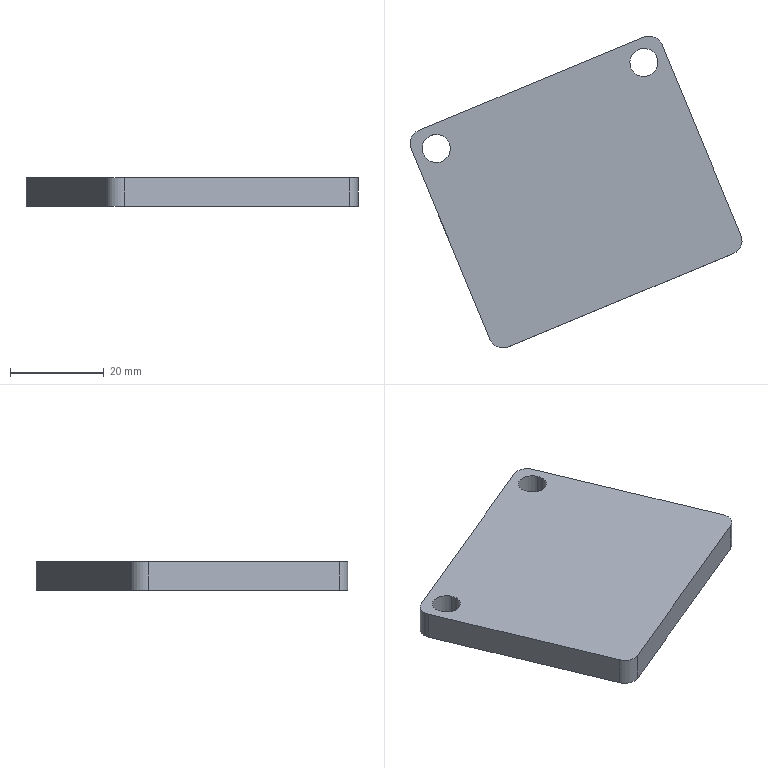Component | SolidWorks | ControlBoard-1 | 1 solid | 14 faces | box 70.89 x 66.56 x 6 mm | volume 17014 mm3 | cylinder 8 | plane 6 | commonest cylinder face diameters 6 x8
build123d program:
from build123d import *

# Parameters (mm, degrees)
SKETCH1_R           = 3
BOSS_EXTRUDE1_DEPTH = 6


with BuildPart() as part:
    # Sketch1 → Boss-Extrude1 (new body)
    with BuildSketch(Plane.XY):
        with BuildLine():
            Line((-18.936, 29.837), (33.064, 29.837))
            ThreePointArc((33.064, 29.837), (35.185, 28.958), (36.064, 26.837))
            Line((36.064, 26.837), (36.064, -17.163))
            ThreePointArc((36.064, -17.163), (35.185, -19.285), (33.064, -20.163))
            Line((33.064, -20.163), (-18.936, -20.163))
            ThreePointArc((-18.936, -20.163), (-21.057, -19.285), (-21.936, -17.163))
            Line((-21.936, -17.163), (-21.936, 26.837))
            ThreePointArc((-21.936, 26.837), (-21.057, 28.958), (-18.936, 29.837))
        make_face()
        with Locations((-16.936, 24.837)):
            Circle(SKETCH1_R, mode=Mode.SUBTRACT)
        with Locations(Location((31.064, 24.837, 0), (0, 0, 180))):
            Circle(SKETCH1_R, mode=Mode.SUBTRACT)
    extrude(amount=BOSS_EXTRUDE1_DEPTH)


solid = part.part

# Placed as in the assembly
solid = solid.moved(Location((28.885, -6.579, 352.846), (0, 0, 22.523)))
STEP:
#1=CARTESIAN_POINT('',(1.783,1.067,14.128));
#2=VERTEX_POINT('',#1);
#3=CARTESIAN_POINT('',(2.001,1.158,14.128));
#4=VERTEX_POINT('',#3);
#5=CARTESIAN_POINT('',(1.892,1.113,14.128));
#6=DIRECTION('',(-0.,0.,1.));
#7=DIRECTION('',(-0.9237,-0.383,0.));
#8=AXIS2_PLACEMENT_3D('',#5,#6,#7);
#9=CIRCLE('',#8,0.1181);
#10=EDGE_CURVE('',#2,#4,#9,.T.);
#11=ORIENTED_EDGE('',*,*,#10,.T.);
#12=CARTESIAN_POINT('',(2.001,1.158,13.892));
#13=VERTEX_POINT('',#12);
#14=CARTESIAN_POINT('',(2.001,1.158,14.128));
#15=DIRECTION('',(0.,-0.,-1.));
#16=VECTOR('',#15,39.37);
#17=LINE('',#14,#16);
#18=EDGE_CURVE('',#4,#13,#17,.T.);
#19=ORIENTED_EDGE('',*,*,#18,.T.);
#20=CARTESIAN_POINT('',(1.783,1.067,13.892));
#21=VERTEX_POINT('',#20);
#22=CARTESIAN_POINT('',(1.892,1.113,13.892));
#23=DIRECTION('',(-0.,0.,1.));
#24=DIRECTION('',(-0.9237,-0.383,0.));
#25=AXIS2_PLACEMENT_3D('',#22,#23,#24);
#26=CIRCLE('',#25,0.1181);
#27=EDGE_CURVE('',#21,#13,#26,.T.);
#28=ORIENTED_EDGE('',*,*,#27,.F.);
#29=CARTESIAN_POINT('',(1.783,1.067,14.128));
#30=DIRECTION('',(0.,-0.,-1.));
#31=VECTOR('',#30,39.37);
#32=LINE('',#29,#31);
#33=EDGE_CURVE('',#2,#21,#32,.T.);
#34=ORIENTED_EDGE('',*,*,#33,.F.);
#35=EDGE_LOOP('',(#11,#19,#28,#34));
#36=FACE_OUTER_BOUND('',#35,.T.);
#37=CARTESIAN_POINT('',(1.892,1.113,14.128));
#38=DIRECTION('',(0.,-0.,-1.));
#39=DIRECTION('',(-0.9237,-0.383,0.));
#40=AXIS2_PLACEMENT_3D('',#37,#38,#39);
#41=CYLINDRICAL_SURFACE('',#40,0.1181);
#42=ADVANCED_FACE('',(#36),#41,.F.);
#43=CARTESIAN_POINT('',(0.03764,0.3436,14.128));
#44=VERTEX_POINT('',#43);
#45=CARTESIAN_POINT('',(0.2558,0.4341,14.128));
#46=VERTEX_POINT('',#45);
#47=CARTESIAN_POINT('',(0.1467,0.3888,14.128));
#48=DIRECTION('',(-0.,0.,1.));
#49=DIRECTION('',(0.9237,0.383,0.));
#50=AXIS2_PLACEMENT_3D('',#47,#48,#49);
#51=CIRCLE('',#50,0.1181);
#52=EDGE_CURVE('',#44,#46,#51,.T.);
#53=ORIENTED_EDGE('',*,*,#52,.T.);
#54=CARTESIAN_POINT('',(0.2558,0.4341,13.892));
#55=VERTEX_POINT('',#54);
#56=CARTESIAN_POINT('',(0.2558,0.4341,14.128));
#57=DIRECTION('',(0.,-0.,-1.));
#58=VECTOR('',#57,39.37);
#59=LINE('',#56,#58);
#60=EDGE_CURVE('',#46,#55,#59,.T.);
#61=ORIENTED_EDGE('',*,*,#60,.T.);
#62=CARTESIAN_POINT('',(0.03764,0.3436,13.892));
#63=VERTEX_POINT('',#62);
#64=CARTESIAN_POINT('',(0.1467,0.3888,13.892));
#65=DIRECTION('',(-0.,0.,1.));
#66=DIRECTION('',(0.9237,0.383,0.));
#67=AXIS2_PLACEMENT_3D('',#64,#65,#66);
#68=CIRCLE('',#67,0.1181);
#69=EDGE_CURVE('',#63,#55,#68,.T.);
#70=ORIENTED_EDGE('',*,*,#69,.F.);
#71=CARTESIAN_POINT('',(0.03764,0.3436,14.128));
#72=DIRECTION('',(0.,-0.,-1.));
#73=VECTOR('',#72,39.37);
#74=LINE('',#71,#73);
#75=EDGE_CURVE('',#44,#63,#74,.T.);
#76=ORIENTED_EDGE('',*,*,#75,.F.);
#77=EDGE_LOOP('',(#53,#61,#70,#76));
#78=FACE_OUTER_BOUND('',#77,.T.);
#79=CARTESIAN_POINT('',(0.1467,0.3888,14.128));
#80=DIRECTION('',(0.,-0.,-1.));
#81=DIRECTION('',(-0.9237,-0.383,0.));
#82=AXIS2_PLACEMENT_3D('',#79,#80,#81);
#83=CYLINDRICAL_SURFACE('',#82,0.1181);
#84=ADVANCED_FACE('',(#78),#83,.F.);
#85=ORIENTED_EDGE('',*,*,#52,.F.);
#86=CARTESIAN_POINT('',(0.1467,0.3888,14.128));
#87=DIRECTION('',(-0.,0.,1.));
#88=DIRECTION('',(0.9237,0.383,0.));
#89=AXIS2_PLACEMENT_3D('',#86,#87,#88);
#90=CIRCLE('',#89,0.1181);
#91=EDGE_CURVE('',#46,#44,#90,.T.);
#92=ORIENTED_EDGE('',*,*,#91,.F.);
#93=EDGE_LOOP('',(#85,#92));
#94=FACE_BOUND('',#93,.T.);
#95=CARTESIAN_POINT('',(2.644,-0.4937,14.128));
#96=VERTEX_POINT('',#95);
#97=CARTESIAN_POINT('',(2.708,-0.3393,14.128));
#98=VERTEX_POINT('',#97);
#99=CARTESIAN_POINT('',(2.598,-0.3846,14.128));
#100=DIRECTION('',(-0.,0.,1.));
#101=DIRECTION('',(0.9237,0.383,0.));
#102=AXIS2_PLACEMENT_3D('',#99,#100,#101);
#103=CIRCLE('',#102,0.1181);
#104=EDGE_CURVE('',#96,#98,#103,.T.);
#105=ORIENTED_EDGE('',*,*,#104,.T.);
#106=CARTESIAN_POINT('',(2.044,1.261,14.128));
#107=VERTEX_POINT('',#106);
#108=CARTESIAN_POINT('',(2.044,1.261,14.128));
#109=DIRECTION('',(-0.383,0.9237,-0.));
#110=VECTOR('',#109,39.37);
#111=LINE('',#108,#110);
#112=EDGE_CURVE('',#98,#107,#111,.T.);
#113=ORIENTED_EDGE('',*,*,#112,.T.);
#114=CARTESIAN_POINT('',(1.89,1.325,14.128));
#115=VERTEX_POINT('',#114);
#116=CARTESIAN_POINT('',(1.935,1.216,14.128));
#117=DIRECTION('',(-0.,0.,1.));
#118=DIRECTION('',(-0.9237,-0.383,0.));
#119=AXIS2_PLACEMENT_3D('',#116,#117,#118);
#120=CIRCLE('',#119,0.1181);
#121=EDGE_CURVE('',#107,#115,#120,.T.);
#122=ORIENTED_EDGE('',*,*,#121,.T.);
#123=CARTESIAN_POINT('',(-0.001396,0.5405,14.128));
#124=VERTEX_POINT('',#123);
#125=CARTESIAN_POINT('',(-0.001396,0.5405,14.128));
#126=DIRECTION('',(-0.9237,-0.383,-0.));
#127=VECTOR('',#126,39.37);
#128=LINE('',#125,#127);
#129=EDGE_CURVE('',#115,#124,#128,.T.);
#130=ORIENTED_EDGE('',*,*,#129,.T.);
#131=CARTESIAN_POINT('',(-0.06526,0.3861,14.128));
#132=VERTEX_POINT('',#131);
#133=CARTESIAN_POINT('',(0.04385,0.4314,14.128));
#134=DIRECTION('',(-0.,0.,1.));
#135=DIRECTION('',(0.9237,0.383,0.));
#136=AXIS2_PLACEMENT_3D('',#133,#134,#135);
#137=CIRCLE('',#136,0.1181);
#138=EDGE_CURVE('',#124,#132,#137,.T.);
#139=ORIENTED_EDGE('',*,*,#138,.T.);
#140=CARTESIAN_POINT('',(0.5983,-1.214,14.128));
#141=VERTEX_POINT('',#140);
#142=CARTESIAN_POINT('',(-0.06526,0.3861,14.128));
#143=DIRECTION('',(0.383,-0.9237,0.));
#144=VECTOR('',#143,39.37);
#145=LINE('',#142,#144);
#146=EDGE_CURVE('',#132,#141,#145,.T.);
#147=ORIENTED_EDGE('',*,*,#146,.T.);
#148=CARTESIAN_POINT('',(0.7526,-1.278,14.128));
#149=VERTEX_POINT('',#148);
#150=CARTESIAN_POINT('',(0.7074,-1.169,14.128));
#151=DIRECTION('',(-0.,0.,1.));
#152=DIRECTION('',(0.9237,0.383,0.));
#153=AXIS2_PLACEMENT_3D('',#150,#151,#152);
#154=CIRCLE('',#153,0.1181);
#155=EDGE_CURVE('',#141,#149,#154,.T.);
#156=ORIENTED_EDGE('',*,*,#155,.T.);
#157=CARTESIAN_POINT('',(0.7526,-1.278,14.128));
#158=DIRECTION('',(0.9237,0.383,0.));
#159=VECTOR('',#158,39.37);
#160=LINE('',#157,#159);
#161=EDGE_CURVE('',#149,#96,#160,.T.);
#162=ORIENTED_EDGE('',*,*,#161,.T.);
#163=EDGE_LOOP('',(#105,#113,#122,#130,#139,#147,#156,#162));
#164=FACE_OUTER_BOUND('',#163,.T.);
#165=ORIENTED_EDGE('',*,*,#10,.F.);
#166=CARTESIAN_POINT('',(1.892,1.113,14.128));
#167=DIRECTION('',(-0.,0.,1.));
#168=DIRECTION('',(-0.9237,-0.383,0.));
#169=AXIS2_PLACEMENT_3D('',#166,#167,#168);
#170=CIRCLE('',#169,0.1181);
#171=EDGE_CURVE('',#4,#2,#170,.T.);
#172=ORIENTED_EDGE('',*,*,#171,.F.);
#173=EDGE_LOOP('',(#165,#172));
#174=FACE_BOUND('',#173,.T.);
#175=CARTESIAN_POINT('',(2.598,-0.3846,14.128));
#176=DIRECTION('',(-0.,0.,1.));
#177=DIRECTION('',(0.9237,0.383,0.));
#178=AXIS2_PLACEMENT_3D('',#175,#176,#177);
#179=PLANE('',#178);
#180=ADVANCED_FACE('',(#94,#164,#174),#179,.T.);
#181=CARTESIAN_POINT('',(2.644,-0.4937,13.892));
#182=VERTEX_POINT('',#181);
#183=CARTESIAN_POINT('',(2.708,-0.3393,13.892));
#184=VERTEX_POINT('',#183);
#185=CARTESIAN_POINT('',(2.598,-0.3846,13.892));
#186=DIRECTION('',(-0.,0.,1.));
#187=DIRECTION('',(0.9237,0.383,0.));
#188=AXIS2_PLACEMENT_3D('',#185,#186,#187);
#189=CIRCLE('',#188,0.1181);
#190=EDGE_CURVE('',#182,#184,#189,.T.);
#191=ORIENTED_EDGE('',*,*,#190,.F.);
#192=CARTESIAN_POINT('',(0.7526,-1.278,13.892));
#193=VERTEX_POINT('',#192);
#194=CARTESIAN_POINT('',(0.7526,-1.278,13.892));
#195=DIRECTION('',(0.9237,0.383,0.));
#196=VECTOR('',#195,39.37);
#197=LINE('',#194,#196);
#198=EDGE_CURVE('',#193,#182,#197,.T.);
#199=ORIENTED_EDGE('',*,*,#198,.F.);
#200=CARTESIAN_POINT('',(0.5983,-1.214,13.892));
#201=VERTEX_POINT('',#200);
#202=CARTESIAN_POINT('',(0.7074,-1.169,13.892));
#203=DIRECTION('',(-0.,0.,1.));
#204=DIRECTION('',(0.9237,0.383,0.));
#205=AXIS2_PLACEMENT_3D('',#202,#203,#204);
#206=CIRCLE('',#205,0.1181);
#207=EDGE_CURVE('',#201,#193,#206,.T.);
#208=ORIENTED_EDGE('',*,*,#207,.F.);
#209=CARTESIAN_POINT('',(-0.06526,0.3861,13.892));
#210=VERTEX_POINT('',#209);
#211=CARTESIAN_POINT('',(-0.06526,0.3861,13.892));
#212=DIRECTION('',(0.383,-0.9237,0.));
#213=VECTOR('',#212,39.37);
#214=LINE('',#211,#213);
#215=EDGE_CURVE('',#210,#201,#214,.T.);
#216=ORIENTED_EDGE('',*,*,#215,.F.);
#217=CARTESIAN_POINT('',(-0.001396,0.5405,13.892));
#218=VERTEX_POINT('',#217);
#219=CARTESIAN_POINT('',(0.04385,0.4314,13.892));
#220=DIRECTION('',(-0.,0.,1.));
#221=DIRECTION('',(0.9237,0.383,0.));
#222=AXIS2_PLACEMENT_3D('',#219,#220,#221);
#223=CIRCLE('',#222,0.1181);
#224=EDGE_CURVE('',#218,#210,#223,.T.);
#225=ORIENTED_EDGE('',*,*,#224,.F.);
#226=CARTESIAN_POINT('',(1.89,1.325,13.892));
#227=VERTEX_POINT('',#226);
#228=CARTESIAN_POINT('',(-0.001396,0.5405,13.892));
#229=DIRECTION('',(-0.9237,-0.383,-0.));
#230=VECTOR('',#229,39.37);
#231=LINE('',#228,#230);
#232=EDGE_CURVE('',#227,#218,#231,.T.);
#233=ORIENTED_EDGE('',*,*,#232,.F.);
#234=CARTESIAN_POINT('',(2.044,1.261,13.892));
#235=VERTEX_POINT('',#234);
#236=CARTESIAN_POINT('',(1.935,1.216,13.892));
#237=DIRECTION('',(-0.,0.,1.));
#238=DIRECTION('',(-0.9237,-0.383,0.));
#239=AXIS2_PLACEMENT_3D('',#236,#237,#238);
#240=CIRCLE('',#239,0.1181);
#241=EDGE_CURVE('',#235,#227,#240,.T.);
#242=ORIENTED_EDGE('',*,*,#241,.F.);
#243=CARTESIAN_POINT('',(2.044,1.261,13.892));
#244=DIRECTION('',(-0.383,0.9237,-0.));
#245=VECTOR('',#244,39.37);
#246=LINE('',#243,#245);
#247=EDGE_CURVE('',#184,#235,#246,.T.);
#248=ORIENTED_EDGE('',*,*,#247,.F.);
#249=EDGE_LOOP('',(#191,#199,#208,#216,#225,#233,#242,#248));
#250=FACE_OUTER_BOUND('',#249,.T.);
#251=ORIENTED_EDGE('',*,*,#69,.T.);
#252=CARTESIAN_POINT('',(0.1467,0.3888,13.892));
#253=DIRECTION('',(-0.,0.,1.));
#254=DIRECTION('',(0.9237,0.383,0.));
#255=AXIS2_PLACEMENT_3D('',#252,#253,#254);
#256=CIRCLE('',#255,0.1181);
#257=EDGE_CURVE('',#55,#63,#256,.T.);
#258=ORIENTED_EDGE('',*,*,#257,.T.);
#259=EDGE_LOOP('',(#251,#258));
#260=FACE_BOUND('',#259,.T.);
#261=ORIENTED_EDGE('',*,*,#27,.T.);
#262=CARTESIAN_POINT('',(1.892,1.113,13.892));
#263=DIRECTION('',(-0.,0.,1.));
#264=DIRECTION('',(-0.9237,-0.383,0.));
#265=AXIS2_PLACEMENT_3D('',#262,#263,#264);
#266=CIRCLE('',#265,0.1181);
#267=EDGE_CURVE('',#13,#21,#266,.T.);
#268=ORIENTED_EDGE('',*,*,#267,.T.);
#269=EDGE_LOOP('',(#261,#268));
#270=FACE_BOUND('',#269,.T.);
#271=CARTESIAN_POINT('',(2.598,-0.3846,13.892));
#272=DIRECTION('',(-0.,0.,1.));
#273=DIRECTION('',(0.9237,0.383,0.));
#274=AXIS2_PLACEMENT_3D('',#271,#272,#273);
#275=PLANE('',#274);
#276=ADVANCED_FACE('',(#250,#260,#270),#275,.F.);
#277=ORIENTED_EDGE('',*,*,#190,.T.);
#278=CARTESIAN_POINT('',(2.708,-0.3393,14.128));
#279=DIRECTION('',(0.,-0.,-1.));
#280=VECTOR('',#279,39.37);
#281=LINE('',#278,#280);
#282=EDGE_CURVE('',#98,#184,#281,.T.);
#283=ORIENTED_EDGE('',*,*,#282,.F.);
#284=ORIENTED_EDGE('',*,*,#104,.F.);
#285=CARTESIAN_POINT('',(2.644,-0.4937,14.128));
#286=DIRECTION('',(0.,-0.,-1.));
#287=VECTOR('',#286,39.37);
#288=LINE('',#285,#287);
#289=EDGE_CURVE('',#96,#182,#288,.T.);
#290=ORIENTED_EDGE('',*,*,#289,.T.);
#291=EDGE_LOOP('',(#277,#283,#284,#290));
#292=FACE_OUTER_BOUND('',#291,.T.);
#293=CARTESIAN_POINT('',(2.598,-0.3846,14.128));
#294=DIRECTION('',(0.,-0.,-1.));
#295=DIRECTION('',(-0.9237,-0.383,0.));
#296=AXIS2_PLACEMENT_3D('',#293,#294,#295);
#297=CYLINDRICAL_SURFACE('',#296,0.1181);
#298=ADVANCED_FACE('',(#292),#297,.T.);
#299=ORIENTED_EDGE('',*,*,#247,.T.);
#300=CARTESIAN_POINT('',(2.044,1.261,14.128));
#301=DIRECTION('',(0.,-0.,-1.));
#302=VECTOR('',#301,39.37);
#303=LINE('',#300,#302);
#304=EDGE_CURVE('',#107,#235,#303,.T.);
#305=ORIENTED_EDGE('',*,*,#304,.F.);
#306=ORIENTED_EDGE('',*,*,#112,.F.);
#307=ORIENTED_EDGE('',*,*,#282,.T.);
#308=EDGE_LOOP('',(#299,#305,#306,#307));
#309=FACE_OUTER_BOUND('',#308,.T.);
#310=CARTESIAN_POINT('',(2.044,1.261,14.128));
#311=DIRECTION('',(-0.9237,-0.383,-0.));
#312=DIRECTION('',(0.383,-0.9237,0.));
#313=AXIS2_PLACEMENT_3D('',#310,#311,#312);
#314=PLANE('',#313);
#315=ADVANCED_FACE('',(#309),#314,.F.);
#316=ORIENTED_EDGE('',*,*,#241,.T.);
#317=CARTESIAN_POINT('',(1.89,1.325,14.128));
#318=DIRECTION('',(0.,-0.,-1.));
#319=VECTOR('',#318,39.37);
#320=LINE('',#317,#319);
#321=EDGE_CURVE('',#115,#227,#320,.T.);
#322=ORIENTED_EDGE('',*,*,#321,.F.);
#323=ORIENTED_EDGE('',*,*,#121,.F.);
#324=ORIENTED_EDGE('',*,*,#304,.T.);
#325=EDGE_LOOP('',(#316,#322,#323,#324));
#326=FACE_OUTER_BOUND('',#325,.T.);
#327=CARTESIAN_POINT('',(1.935,1.216,14.128));
#328=DIRECTION('',(0.,-0.,-1.));
#329=DIRECTION('',(-0.9237,-0.383,0.));
#330=AXIS2_PLACEMENT_3D('',#327,#328,#329);
#331=CYLINDRICAL_SURFACE('',#330,0.1181);
#332=ADVANCED_FACE('',(#326),#331,.T.);
#333=ORIENTED_EDGE('',*,*,#232,.T.);
#334=CARTESIAN_POINT('',(-0.001396,0.5405,14.128));
#335=DIRECTION('',(0.,-0.,-1.));
#336=VECTOR('',#335,39.37);
#337=LINE('',#334,#336);
#338=EDGE_CURVE('',#124,#218,#337,.T.);
#339=ORIENTED_EDGE('',*,*,#338,.F.);
#340=ORIENTED_EDGE('',*,*,#129,.F.);
#341=ORIENTED_EDGE('',*,*,#321,.T.);
#342=EDGE_LOOP('',(#333,#339,#340,#341));
#343=FACE_OUTER_BOUND('',#342,.T.);
#344=CARTESIAN_POINT('',(-0.001396,0.5405,14.128));
#345=DIRECTION('',(0.383,-0.9237,0.));
#346=DIRECTION('',(0.,-0.,-1.));
#347=AXIS2_PLACEMENT_3D('',#344,#345,#346);
#348=PLANE('',#347);
#349=ADVANCED_FACE('',(#343),#348,.F.);
#350=ORIENTED_EDGE('',*,*,#224,.T.);
#351=CARTESIAN_POINT('',(-0.06526,0.3861,14.128));
#352=DIRECTION('',(0.,-0.,-1.));
#353=VECTOR('',#352,39.37);
#354=LINE('',#351,#353);
#355=EDGE_CURVE('',#132,#210,#354,.T.);
#356=ORIENTED_EDGE('',*,*,#355,.F.);
#357=ORIENTED_EDGE('',*,*,#138,.F.);
#358=ORIENTED_EDGE('',*,*,#338,.T.);
#359=EDGE_LOOP('',(#350,#356,#357,#358));
#360=FACE_OUTER_BOUND('',#359,.T.);
#361=CARTESIAN_POINT('',(0.04385,0.4314,14.128));
#362=DIRECTION('',(0.,-0.,-1.));
#363=DIRECTION('',(-0.9237,-0.383,0.));
#364=AXIS2_PLACEMENT_3D('',#361,#362,#363);
#365=CYLINDRICAL_SURFACE('',#364,0.1181);
#366=ADVANCED_FACE('',(#360),#365,.T.);
#367=ORIENTED_EDGE('',*,*,#215,.T.);
#368=CARTESIAN_POINT('',(0.5983,-1.214,14.128));
#369=DIRECTION('',(0.,-0.,-1.));
#370=VECTOR('',#369,39.37);
#371=LINE('',#368,#370);
#372=EDGE_CURVE('',#141,#201,#371,.T.);
#373=ORIENTED_EDGE('',*,*,#372,.F.);
#374=ORIENTED_EDGE('',*,*,#146,.F.);
#375=ORIENTED_EDGE('',*,*,#355,.T.);
#376=EDGE_LOOP('',(#367,#373,#374,#375));
#377=FACE_OUTER_BOUND('',#376,.T.);
#378=CARTESIAN_POINT('',(-0.06526,0.3861,14.128));
#379=DIRECTION('',(0.9237,0.383,0.));
#380=DIRECTION('',(-0.383,0.9237,-0.));
#381=AXIS2_PLACEMENT_3D('',#378,#379,#380);
#382=PLANE('',#381);
#383=ADVANCED_FACE('',(#377),#382,.F.);
#384=ORIENTED_EDGE('',*,*,#207,.T.);
#385=CARTESIAN_POINT('',(0.7526,-1.278,14.128));
#386=DIRECTION('',(0.,-0.,-1.));
#387=VECTOR('',#386,39.37);
#388=LINE('',#385,#387);
#389=EDGE_CURVE('',#149,#193,#388,.T.);
#390=ORIENTED_EDGE('',*,*,#389,.F.);
#391=ORIENTED_EDGE('',*,*,#155,.F.);
#392=ORIENTED_EDGE('',*,*,#372,.T.);
#393=EDGE_LOOP('',(#384,#390,#391,#392));
#394=FACE_OUTER_BOUND('',#393,.T.);
#395=CARTESIAN_POINT('',(0.7074,-1.169,14.128));
#396=DIRECTION('',(0.,-0.,-1.));
#397=DIRECTION('',(-0.9237,-0.383,0.));
#398=AXIS2_PLACEMENT_3D('',#395,#396,#397);
#399=CYLINDRICAL_SURFACE('',#398,0.1181);
#400=ADVANCED_FACE('',(#394),#399,.T.);
#401=ORIENTED_EDGE('',*,*,#198,.T.);
#402=ORIENTED_EDGE('',*,*,#289,.F.);
#403=ORIENTED_EDGE('',*,*,#161,.F.);
#404=ORIENTED_EDGE('',*,*,#389,.T.);
#405=EDGE_LOOP('',(#401,#402,#403,#404));
#406=FACE_OUTER_BOUND('',#405,.T.);
#407=CARTESIAN_POINT('',(0.7526,-1.278,14.128));
#408=DIRECTION('',(-0.383,0.9237,-0.));
#409=DIRECTION('',(-0.,0.,1.));
#410=AXIS2_PLACEMENT_3D('',#407,#408,#409);
#411=PLANE('',#410);
#412=ADVANCED_FACE('',(#406),#411,.F.);
#413=ORIENTED_EDGE('',*,*,#60,.F.);
#414=ORIENTED_EDGE('',*,*,#91,.T.);
#415=ORIENTED_EDGE('',*,*,#75,.T.);
#416=ORIENTED_EDGE('',*,*,#257,.F.);
#417=EDGE_LOOP('',(#413,#414,#415,#416));
#418=FACE_OUTER_BOUND('',#417,.T.);
#419=CARTESIAN_POINT('',(0.1467,0.3888,14.128));
#420=DIRECTION('',(0.,-0.,-1.));
#421=DIRECTION('',(-0.9237,-0.383,0.));
#422=AXIS2_PLACEMENT_3D('',#419,#420,#421);
#423=CYLINDRICAL_SURFACE('',#422,0.1181);
#424=ADVANCED_FACE('',(#418),#423,.F.);
#425=ORIENTED_EDGE('',*,*,#18,.F.);
#426=ORIENTED_EDGE('',*,*,#171,.T.);
#427=ORIENTED_EDGE('',*,*,#33,.T.);
#428=ORIENTED_EDGE('',*,*,#267,.F.);
#429=EDGE_LOOP('',(#425,#426,#427,#428));
#430=FACE_OUTER_BOUND('',#429,.T.);
#431=CARTESIAN_POINT('',(1.892,1.113,14.128));
#432=DIRECTION('',(0.,-0.,-1.));
#433=DIRECTION('',(-0.9237,-0.383,0.));
#434=AXIS2_PLACEMENT_3D('',#431,#432,#433);
#435=CYLINDRICAL_SURFACE('',#434,0.1181);
#436=ADVANCED_FACE('',(#430),#435,.F.);
#437=CLOSED_SHELL('',(#42,#84,#180,#276,#298,#315,#332,#349,#366,#383,#400,#412,#424,#436));
#438=MANIFOLD_SOLID_BREP('',#437);
#439=CARTESIAN_POINT('',(0.,0.,0.));
#440=DIRECTION('',(0.,0.,1.));
#441=DIRECTION('',(1.,0.,0.));
#442=AXIS2_PLACEMENT_3D('',#439,#440,#441);
#443=(LENGTH_UNIT()NAMED_UNIT(*)SI_UNIT($,.METRE.));
#444=LENGTH_MEASURE_WITH_UNIT(LENGTH_MEASURE(0.0254),#443);
#445=DIMENSIONAL_EXPONENTS(1.,0.,0.,0.,0.,0.,0.);
#446=(CONVERSION_BASED_UNIT('',#444)LENGTH_UNIT()NAMED_UNIT(#445));
#447=UNCERTAINTY_MEASURE_WITH_UNIT(LENGTH_MEASURE(0.00001),#446,'','');
#448=(NAMED_UNIT(*)PLANE_ANGLE_UNIT()SI_UNIT($,.RADIAN.));
#449=(NAMED_UNIT(*)SI_UNIT($,.STERADIAN.)SOLID_ANGLE_UNIT());
#450=(GEOMETRIC_REPRESENTATION_CONTEXT(3)GLOBAL_UNCERTAINTY_ASSIGNED_CONTEXT((#447))GLOBAL_UNIT_ASSIGNED_CONTEXT((#446,#448,#449))REPRESENTATION_CONTEXT('',''));
#451=ADVANCED_BREP_SHAPE_REPRESENTATION('',(#438,#442),#450);
#452=COLOUR_RGB('',0.7922,0.8196,0.9333);
#453=FILL_AREA_STYLE_COLOUR('',#452);
#454=FILL_AREA_STYLE('',(#453));
#455=SURFACE_STYLE_FILL_AREA(#454);
#456=SURFACE_SIDE_STYLE('',(#455));
#457=SURFACE_STYLE_USAGE(.BOTH.,#456);
#458=PRESENTATION_STYLE_ASSIGNMENT((#457));
#459=STYLED_ITEM('',(#458),#438);
#460=(LENGTH_UNIT()NAMED_UNIT(*)SI_UNIT($,.METRE.));
#461=LENGTH_MEASURE_WITH_UNIT(LENGTH_MEASURE(0.0254),#460);
#462=DIMENSIONAL_EXPONENTS(1.,0.,0.,0.,0.,0.,0.);
#463=(CONVERSION_BASED_UNIT('',#461)LENGTH_UNIT()NAMED_UNIT(#462));
#464=UNCERTAINTY_MEASURE_WITH_UNIT(LENGTH_MEASURE(0.00001),#463,'','');
#465=(NAMED_UNIT(*)PLANE_ANGLE_UNIT()SI_UNIT($,.RADIAN.));
#466=(NAMED_UNIT(*)SI_UNIT($,.STERADIAN.)SOLID_ANGLE_UNIT());
#467=(GEOMETRIC_REPRESENTATION_CONTEXT(3)GLOBAL_UNCERTAINTY_ASSIGNED_CONTEXT((#464))GLOBAL_UNIT_ASSIGNED_CONTEXT((#463,#465,#466))REPRESENTATION_CONTEXT('',''));
#468=MECHANICAL_DESIGN_GEOMETRIC_PRESENTATION_REPRESENTATION('',(#459),#467);
#469=PRESENTATION_LAYER_ASSIGNMENT('','',(#459));